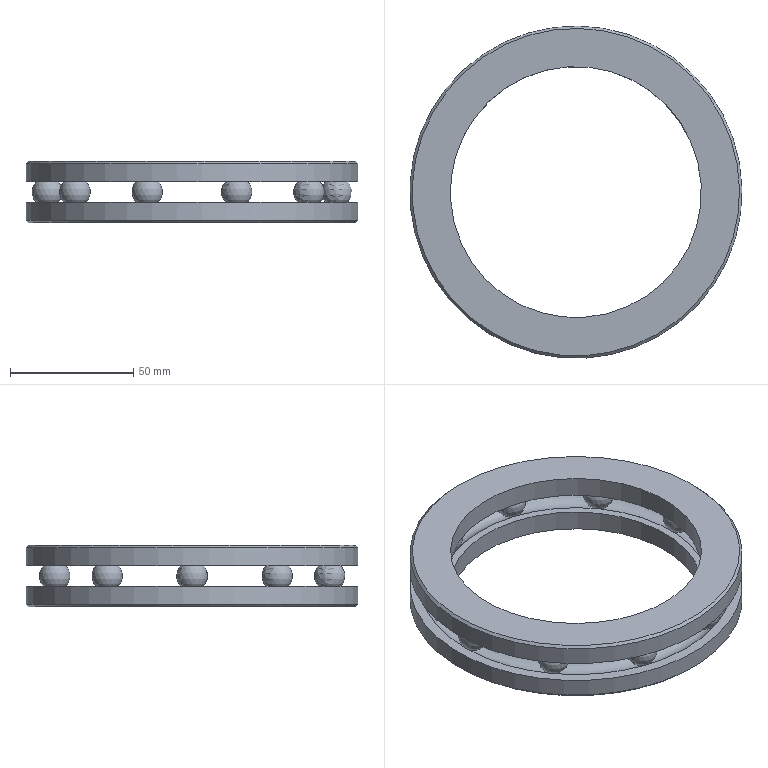Component | NX | CA6140-ZHUZHOU-D8120 | 12 solids | 24 faces | volume 102075 mm3 | sphere 10 | plane 6 | cylinder 4 | cone 2 | torus 2 | commonest cylinder face diameters 135 x2 102 x2